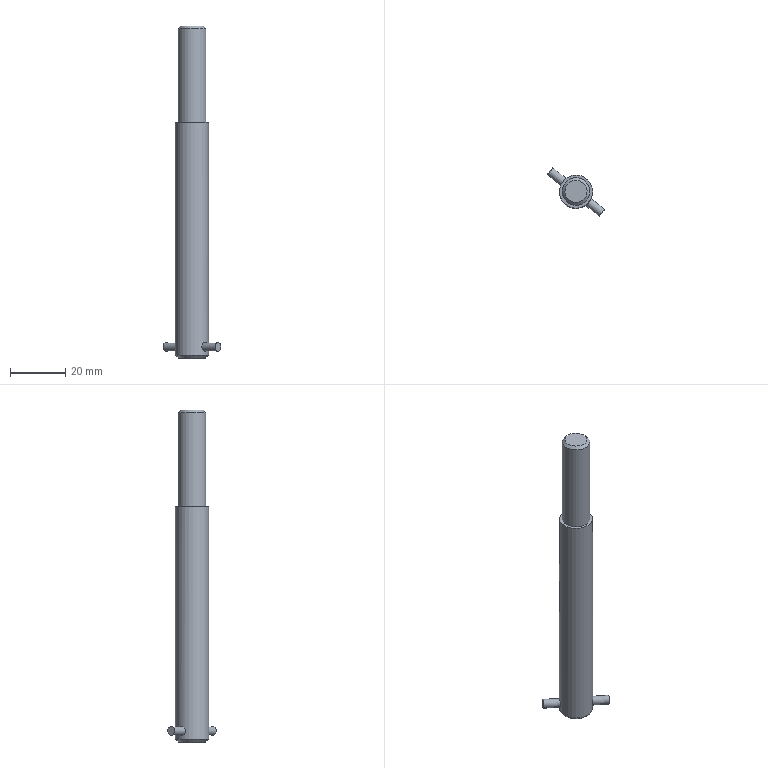Component | NX | PIN_FOR_SPRING | 2 solids | 11 faces | volume 12427 mm3 | plane 5 | cylinder 4 | cone 2 | commonest cylinder face diameters 3.2 x2 12 x1 10 x1